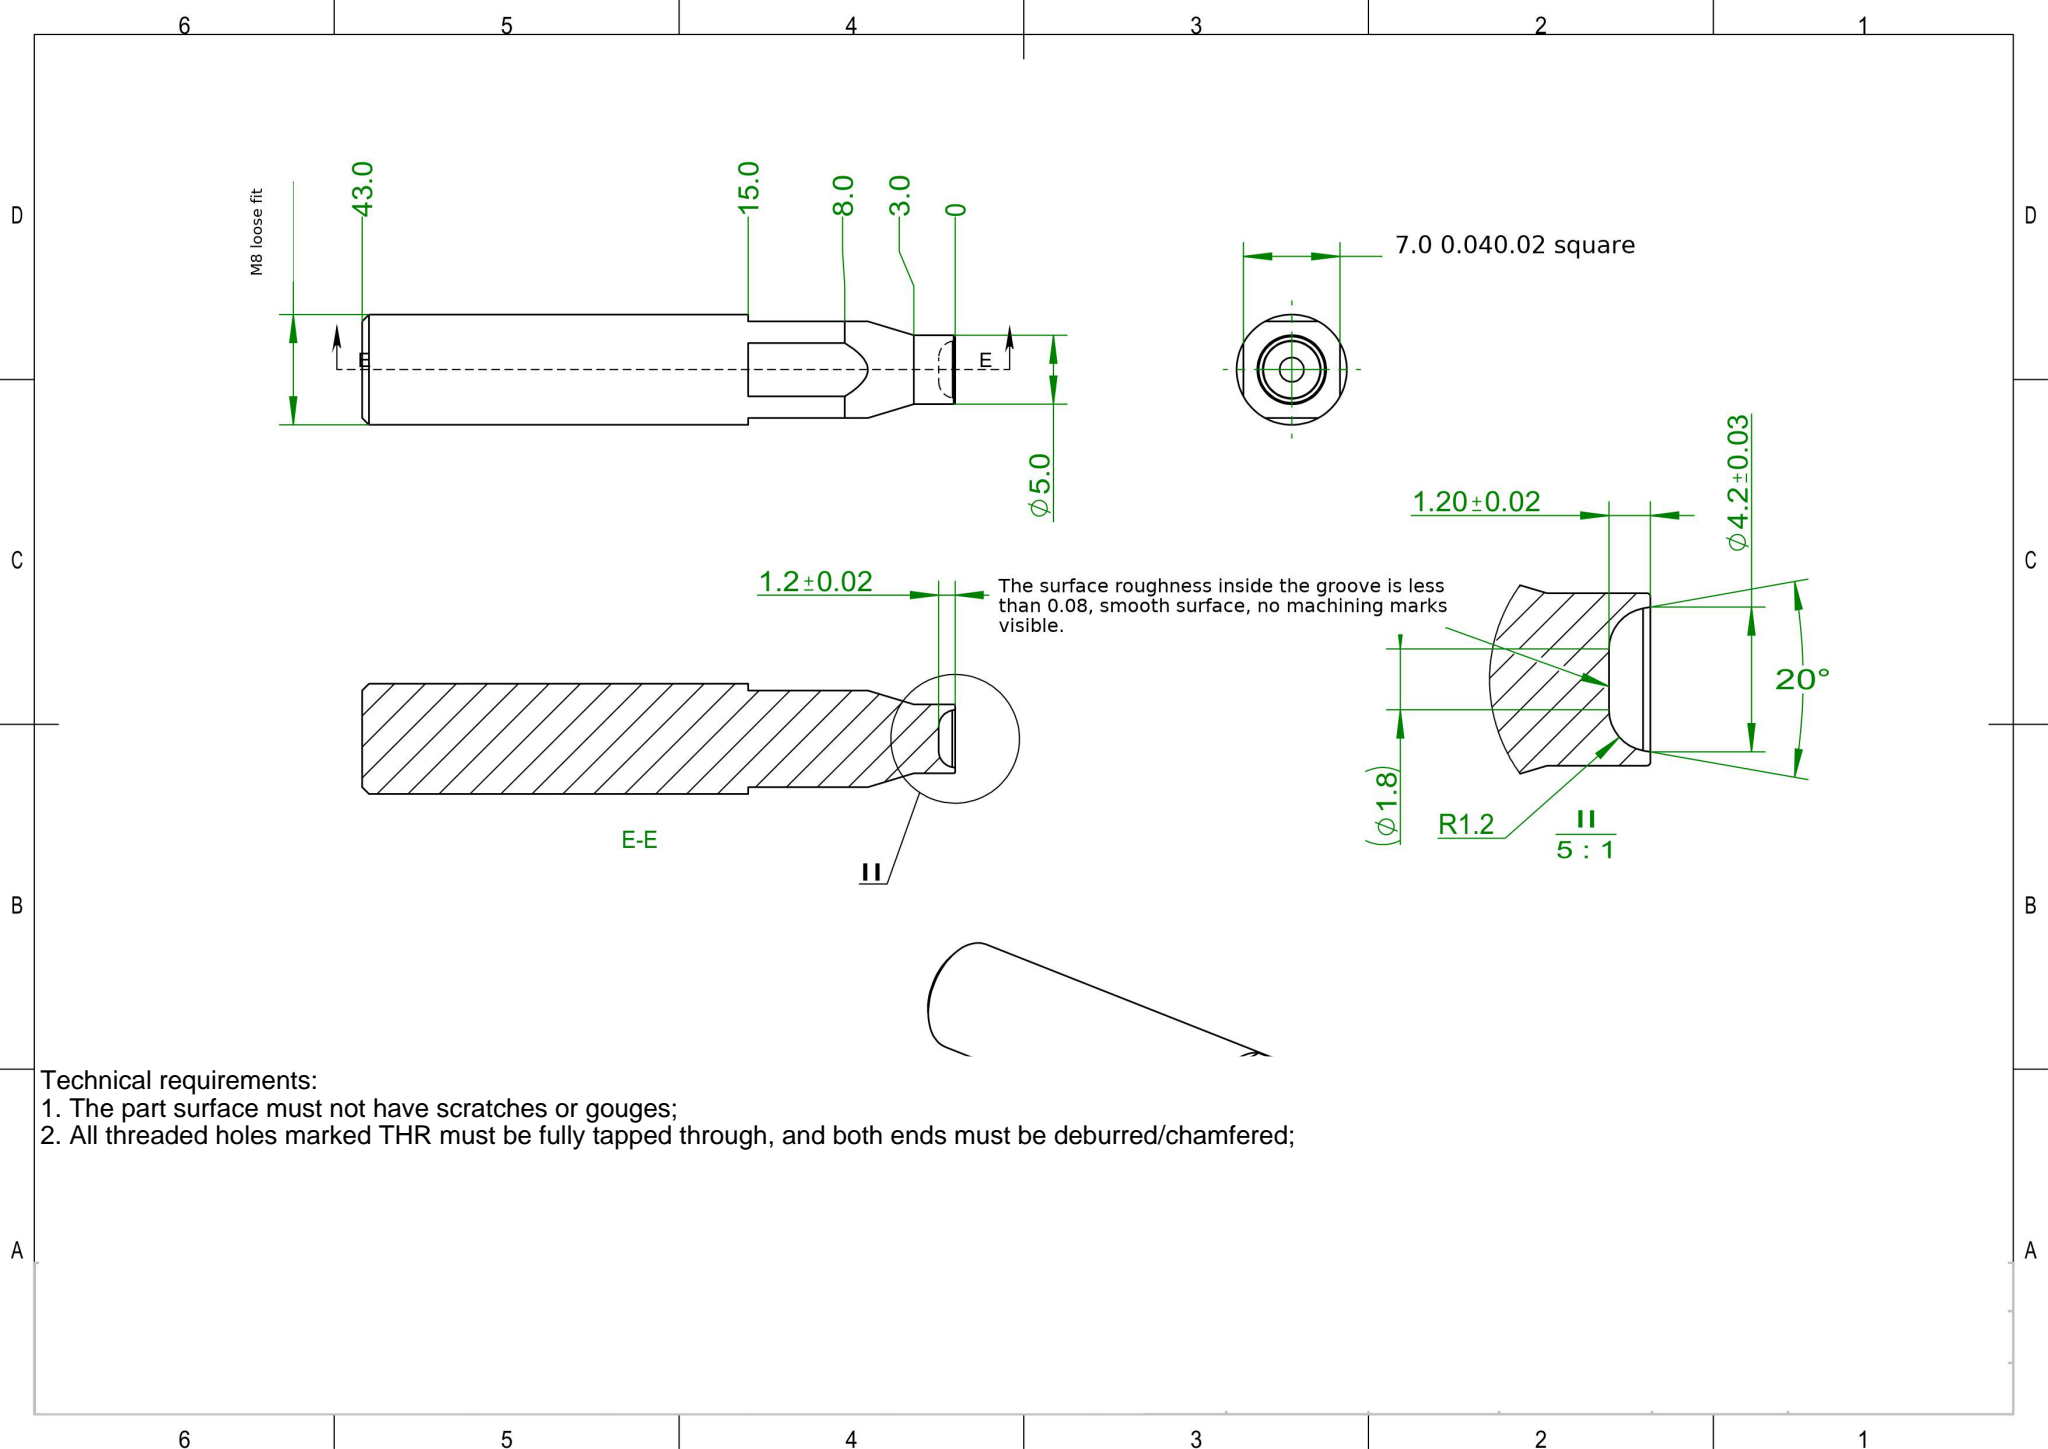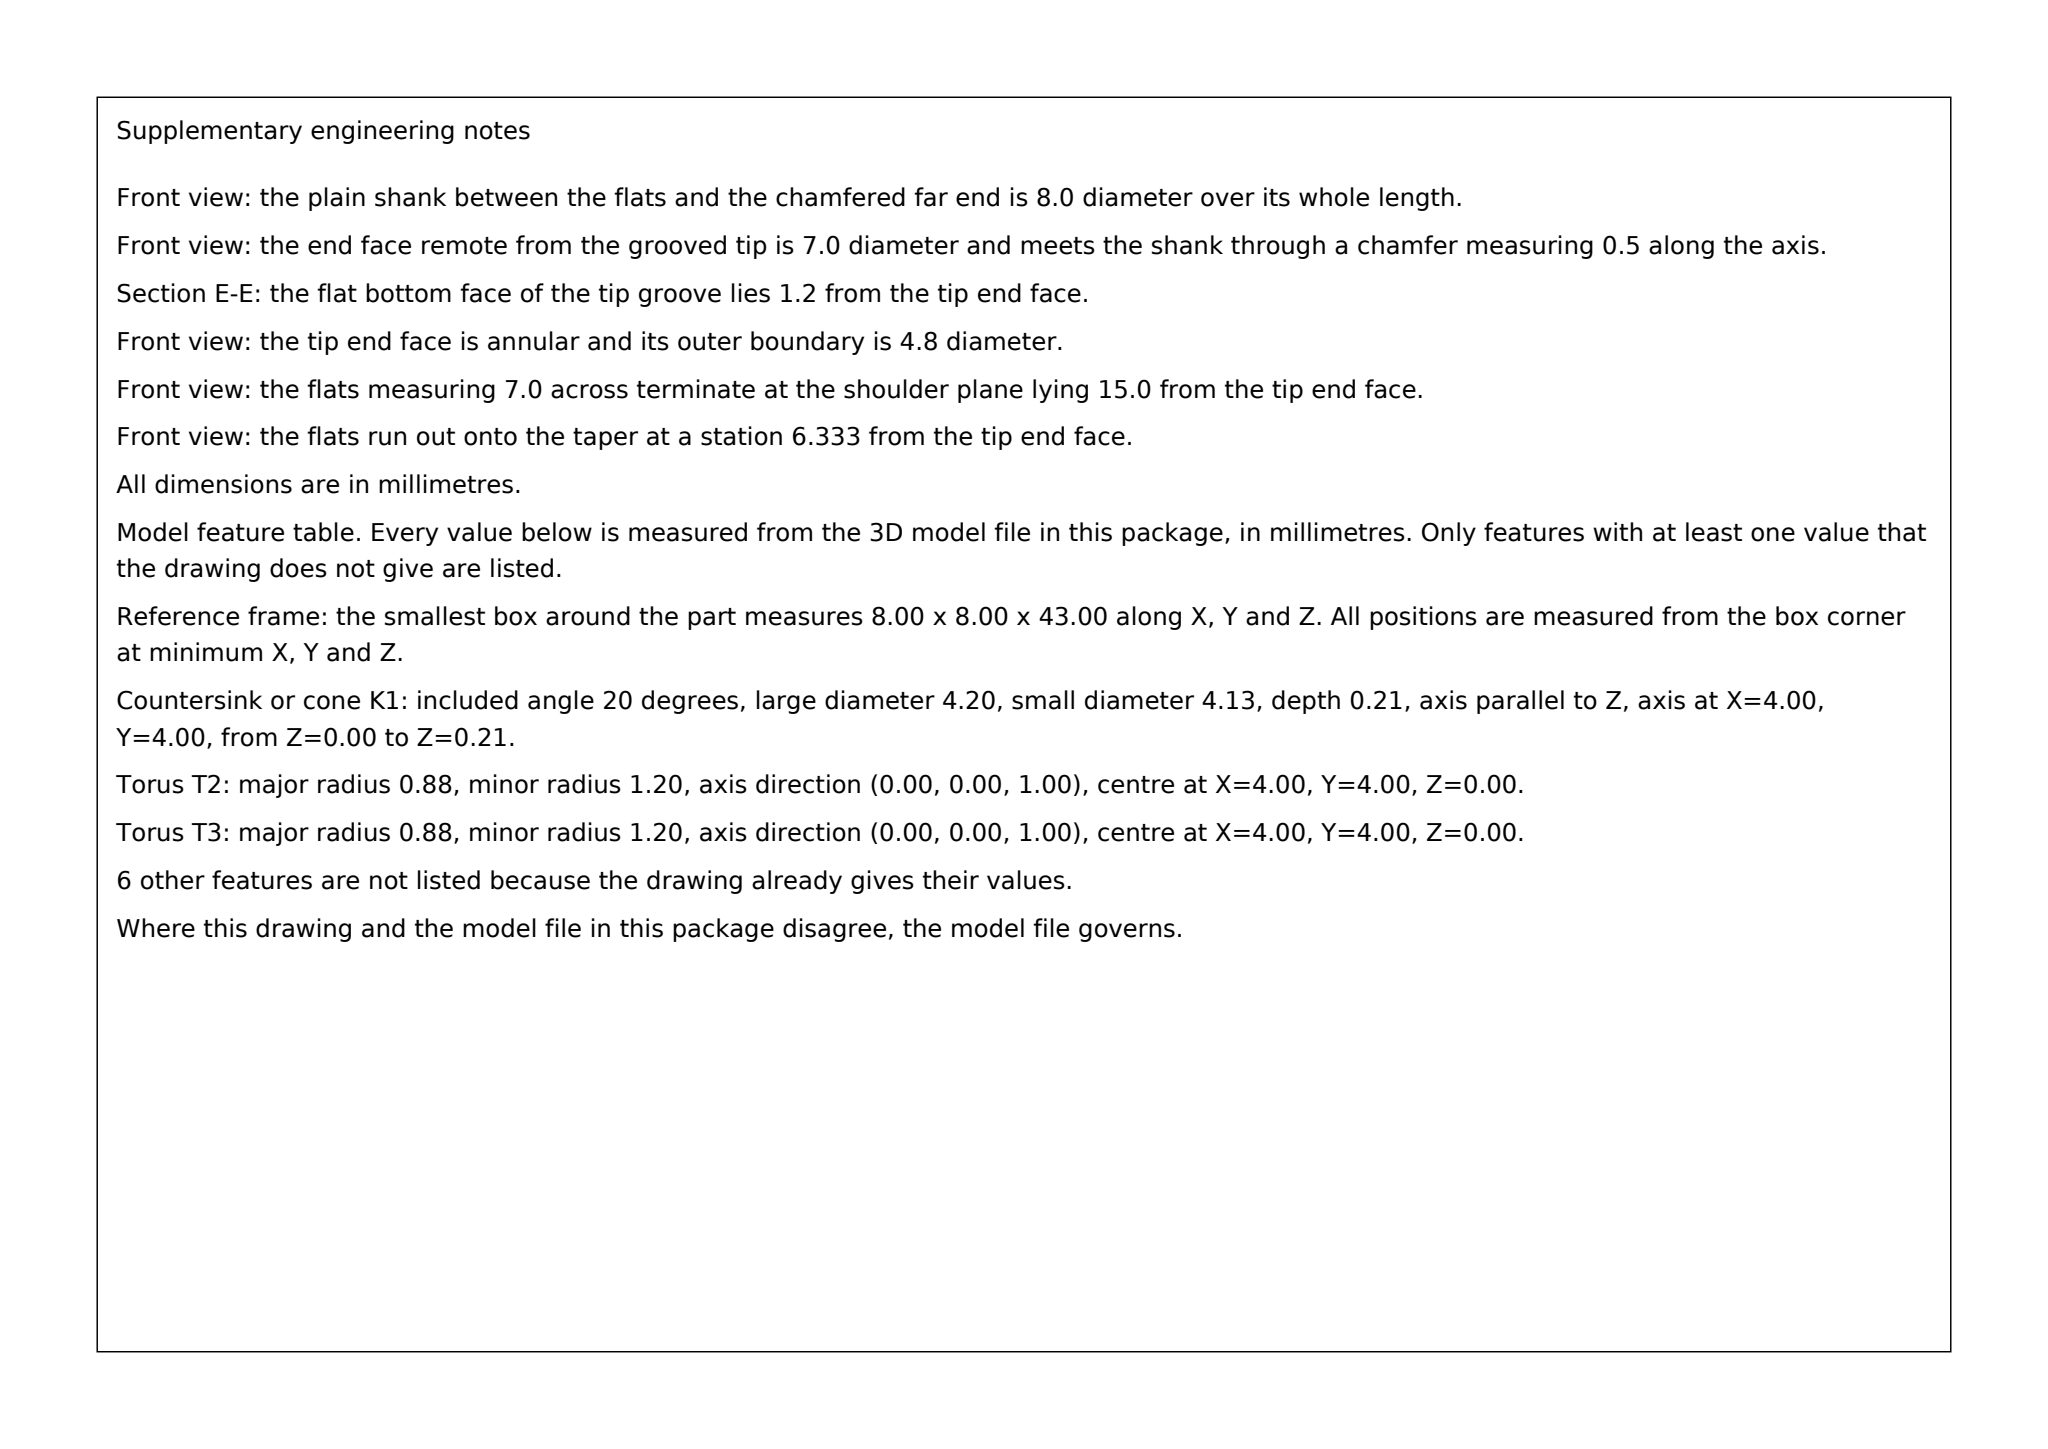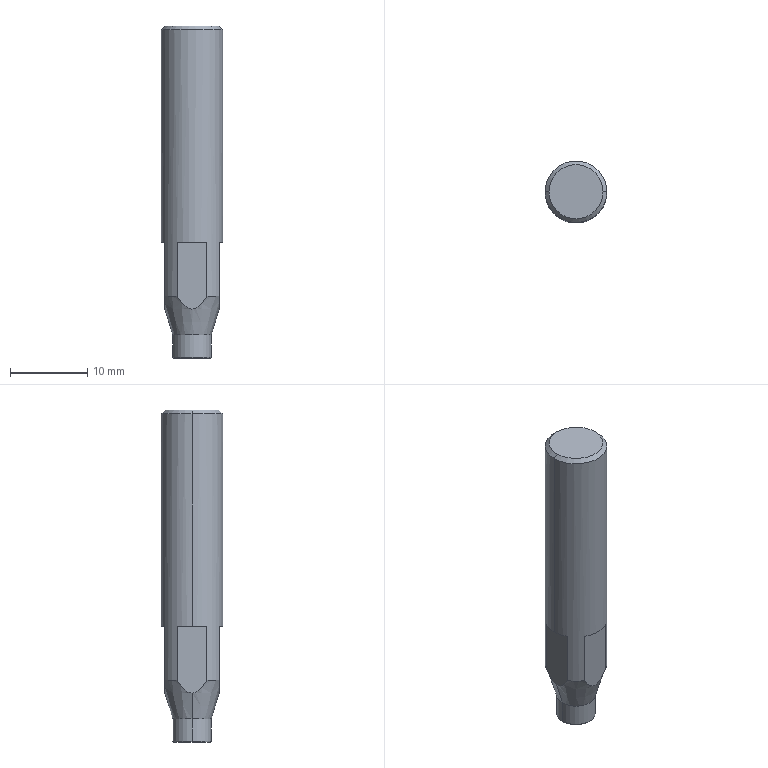Part | SolidWorks | mm | 1 solid | 25 faces | box 8 x 8 x 43 mm | volume 1931 mm3 | plane 11 | cone 6 | torus 4 | cylinder 4 | commonest cylinder face diameters 5 x2 8 x2
Drawing notes:
MAIN BODY OD Ø8.0, ORD 8.0 TO 43.0 (34.5 LG) | from the solid: cylinder [8.0 dia, z axis, 34.5 long] on axis x=4,y=4
TAPER 33.4° INCL, Ø8.0 TO Ø5.0, ORD 8.0 TO 3.0 | from the solid: cone [included 33.4°, ref dia 8.0]; Ø5 and Ø8 cylinders coaxial
R0.1 FILLETS (2) AT Ø5.0 NOSE TRANSITION | from the solid: fillet_radii [0.1, count 2]
DETAIL II: GROOVE FLAT BOT Ø1.76 AT 1.2 DP, BLEND R1.2 | from the solid: Plane z=1.2 (groove bottom) + cone incl 20° ref Ø4.2 at z=0 face + fillet R1.2: Ø4.2-2(1.2)tan10°=Ø3.777 at bottom, less 2x(1.2/tan50°)=2.014 -> Ø1.76 flat (shown Ø1.8 ref)
SQUARE DRIVE FLATS: 7.0 ACROSS FLATS (TWO PAIRS AT 90°), SYMMETRIC ABOUT PART AXIS ON Ø8.0 BODY; FLAT ENDS AT Z=15.0 FROM NOSE END (Z=0) | from the solid: axis_planes x@0.5 & x@7.5, y@0.5 & y@7.5 (8.0 bbox -> 7.0 across flats); axis_planes z@15.0 (4 faces)
SQUARE DRIVE FLAT RUN-OUT: 90° INCLUDED ANGLE CONE, REF Ø7.0, AT FLAT TERMINATION Z=15.0 FROM NOSE END (Z=0), COAXIAL WITH PART AXIS | from the solid: cones[included_angle,ref_dia] = [90.0, 7.0, 2]; axis_planes z offset 15.0 (count 4)
STEP:
#1=CARTESIAN_POINT('',(-2.063,0.,-1.792));
#2=VERTEX_POINT('',#1);
#3=CARTESIAN_POINT('',(2.063,0.,-1.792));
#4=VERTEX_POINT('',#3);
#5=CARTESIAN_POINT('',(0.,0.,-1.792));
#6=DIRECTION('',(0.,0.,1.));
#7=DIRECTION('',(-1.,0.,0.));
#8=AXIS2_PLACEMENT_3D('',#5,#6,#7);
#9=CIRCLE('',#8,2.063);
#10=EDGE_CURVE('',#2,#4,#9,.T.);
#11=ORIENTED_EDGE('',*,*,#10,.F.);
#12=CARTESIAN_POINT('',(-0.8815,0.,-0.8));
#13=VERTEX_POINT('',#12);
#14=CARTESIAN_POINT('',(-0.8815,0.,-2.));
#15=DIRECTION('',(0.,1.,0.));
#16=DIRECTION('',(-1.,0.,0.));
#17=AXIS2_PLACEMENT_3D('',#14,#15,#16);
#18=CIRCLE('',#17,1.2);
#19=EDGE_CURVE('',#2,#13,#18,.T.);
#20=ORIENTED_EDGE('',*,*,#19,.T.);
#21=CARTESIAN_POINT('',(0.8815,0.,-0.8));
#22=VERTEX_POINT('',#21);
#23=CARTESIAN_POINT('',(0.,0.,-0.8));
#24=DIRECTION('',(0.,0.,-1.));
#25=DIRECTION('',(1.,0.,0.));
#26=AXIS2_PLACEMENT_3D('',#23,#24,#25);
#27=CIRCLE('',#26,0.8815);
#28=EDGE_CURVE('',#22,#13,#27,.T.);
#29=ORIENTED_EDGE('',*,*,#28,.F.);
#30=CARTESIAN_POINT('',(0.8815,0.,-2.));
#31=DIRECTION('',(0.,-1.,0.));
#32=DIRECTION('',(0.,0.,-1.));
#33=AXIS2_PLACEMENT_3D('',#30,#31,#32);
#34=CIRCLE('',#33,1.2);
#35=EDGE_CURVE('',#4,#22,#34,.T.);
#36=ORIENTED_EDGE('',*,*,#35,.F.);
#37=EDGE_LOOP('',(#11,#20,#29,#36));
#38=FACE_OUTER_BOUND('',#37,.T.);
#39=CARTESIAN_POINT('',(0.,0.,-2.));
#40=DIRECTION('',(0.,0.,1.));
#41=DIRECTION('',(1.,0.,0.));
#42=AXIS2_PLACEMENT_3D('',#39,#40,#41);
#43=TOROIDAL_SURFACE('',#42,0.8815,1.2);
#44=ADVANCED_FACE('',(#38),#43,.F.);
#45=ORIENTED_EDGE('',*,*,#10,.T.);
#46=CARTESIAN_POINT('',(2.1,0.,-2.));
#47=VERTEX_POINT('',#46);
#48=CARTESIAN_POINT('',(2.1,0.,-2.));
#49=DIRECTION('',(0.1736,0.,-0.9848));
#50=VECTOR('',#49,1000.);
#51=LINE('',#48,#50);
#52=EDGE_CURVE('',#4,#47,#51,.T.);
#53=ORIENTED_EDGE('',*,*,#52,.T.);
#54=CARTESIAN_POINT('',(-2.1,0.,-2.));
#55=VERTEX_POINT('',#54);
#56=CARTESIAN_POINT('',(0.,0.,-2.));
#57=DIRECTION('',(0.,0.,-1.));
#58=DIRECTION('',(-1.,0.,0.));
#59=AXIS2_PLACEMENT_3D('',#56,#57,#58);
#60=CIRCLE('',#59,2.1);
#61=EDGE_CURVE('',#47,#55,#60,.T.);
#62=ORIENTED_EDGE('',*,*,#61,.T.);
#63=CARTESIAN_POINT('',(-2.1,0.,-2.));
#64=DIRECTION('',(-0.1736,0.,-0.9848));
#65=VECTOR('',#64,1000.);
#66=LINE('',#63,#65);
#67=EDGE_CURVE('',#2,#55,#66,.T.);
#68=ORIENTED_EDGE('',*,*,#67,.F.);
#69=EDGE_LOOP('',(#45,#53,#62,#68));
#70=FACE_OUTER_BOUND('',#69,.T.);
#71=CARTESIAN_POINT('',(0.,0.,-2.));
#72=DIRECTION('',(0.,0.,-1.));
#73=DIRECTION('',(-1.,0.,0.));
#74=AXIS2_PLACEMENT_3D('',#71,#72,#73);
#75=CONICAL_SURFACE('',#74,2.1,0.1745);
#76=ADVANCED_FACE('',(#70),#75,.F.);
#77=CARTESIAN_POINT('',(3.5,0.,41.));
#78=VERTEX_POINT('',#77);
#79=CARTESIAN_POINT('',(-3.5,0.,41.));
#80=VERTEX_POINT('',#79);
#81=CARTESIAN_POINT('',(0.,0.,41.));
#82=DIRECTION('',(0.,0.,1.));
#83=DIRECTION('',(1.,0.,0.));
#84=AXIS2_PLACEMENT_3D('',#81,#82,#83);
#85=CIRCLE('',#84,3.5);
#86=EDGE_CURVE('',#78,#80,#85,.T.);
#87=ORIENTED_EDGE('',*,*,#86,.F.);
#88=CARTESIAN_POINT('',(4.,0.,40.5));
#89=VERTEX_POINT('',#88);
#90=CARTESIAN_POINT('',(3.5,0.,41.));
#91=DIRECTION('',(0.7071,0.,-0.7071));
#92=VECTOR('',#91,1000.);
#93=LINE('',#90,#92);
#94=EDGE_CURVE('',#78,#89,#93,.T.);
#95=ORIENTED_EDGE('',*,*,#94,.T.);
#96=CARTESIAN_POINT('',(-4.,0.,40.5));
#97=VERTEX_POINT('',#96);
#98=CARTESIAN_POINT('',(0.,0.,40.5));
#99=DIRECTION('',(0.,0.,-1.));
#100=DIRECTION('',(1.,0.,0.));
#101=AXIS2_PLACEMENT_3D('',#98,#99,#100);
#102=CIRCLE('',#101,4.);
#103=EDGE_CURVE('',#97,#89,#102,.T.);
#104=ORIENTED_EDGE('',*,*,#103,.F.);
#105=CARTESIAN_POINT('',(-3.5,0.,41.));
#106=DIRECTION('',(-0.7071,0.,-0.7071));
#107=VECTOR('',#106,1000.);
#108=LINE('',#105,#107);
#109=EDGE_CURVE('',#80,#97,#108,.T.);
#110=ORIENTED_EDGE('',*,*,#109,.F.);
#111=EDGE_LOOP('',(#87,#95,#104,#110));
#112=FACE_OUTER_BOUND('',#111,.T.);
#113=CARTESIAN_POINT('',(0.,0.,41.));
#114=DIRECTION('',(0.,0.,-1.));
#115=DIRECTION('',(-1.,0.,0.));
#116=AXIS2_PLACEMENT_3D('',#113,#114,#115);
#117=CONICAL_SURFACE('',#116,3.5,0.7854);
#118=ADVANCED_FACE('',(#112),#117,.T.);
#119=CARTESIAN_POINT('',(2.5,0.,1.));
#120=VERTEX_POINT('',#119);
#121=CARTESIAN_POINT('',(-2.5,0.,1.));
#122=VERTEX_POINT('',#121);
#123=CARTESIAN_POINT('',(0.,0.,1.));
#124=DIRECTION('',(0.,0.,1.));
#125=DIRECTION('',(1.,0.,0.));
#126=AXIS2_PLACEMENT_3D('',#123,#124,#125);
#127=CIRCLE('',#126,2.5);
#128=EDGE_CURVE('',#120,#122,#127,.T.);
#129=ORIENTED_EDGE('',*,*,#128,.F.);
#130=CARTESIAN_POINT('',(2.5,0.,-1.9));
#131=VERTEX_POINT('',#130);
#132=CARTESIAN_POINT('',(2.5,0.,11.5));
#133=DIRECTION('',(0.,0.,-1.));
#134=VECTOR('',#133,1000.);
#135=LINE('',#132,#134);
#136=EDGE_CURVE('',#120,#131,#135,.T.);
#137=ORIENTED_EDGE('',*,*,#136,.T.);
#138=CARTESIAN_POINT('',(-2.5,0.,-1.9));
#139=VERTEX_POINT('',#138);
#140=CARTESIAN_POINT('',(0.,0.,-1.9));
#141=DIRECTION('',(0.,0.,1.));
#142=DIRECTION('',(1.,0.,0.));
#143=AXIS2_PLACEMENT_3D('',#140,#141,#142);
#144=CIRCLE('',#143,2.5);
#145=EDGE_CURVE('',#131,#139,#144,.T.);
#146=ORIENTED_EDGE('',*,*,#145,.T.);
#147=CARTESIAN_POINT('',(-2.5,0.,11.5));
#148=DIRECTION('',(0.,0.,-1.));
#149=VECTOR('',#148,1000.);
#150=LINE('',#147,#149);
#151=EDGE_CURVE('',#122,#139,#150,.T.);
#152=ORIENTED_EDGE('',*,*,#151,.F.);
#153=EDGE_LOOP('',(#129,#137,#146,#152));
#154=FACE_OUTER_BOUND('',#153,.T.);
#155=CARTESIAN_POINT('',(0.,0.,11.5));
#156=DIRECTION('',(0.,0.,-1.));
#157=DIRECTION('',(-1.,0.,0.));
#158=AXIS2_PLACEMENT_3D('',#155,#156,#157);
#159=CYLINDRICAL_SURFACE('',#158,2.5);
#160=ADVANCED_FACE('',(#154),#159,.T.);
#161=CARTESIAN_POINT('',(-2.4,0.,-2.));
#162=VERTEX_POINT('',#161);
#163=CARTESIAN_POINT('',(2.4,0.,-2.));
#164=VERTEX_POINT('',#163);
#165=CARTESIAN_POINT('',(0.,0.,-2.));
#166=DIRECTION('',(0.,0.,-1.));
#167=DIRECTION('',(1.,0.,0.));
#168=AXIS2_PLACEMENT_3D('',#165,#166,#167);
#169=CIRCLE('',#168,2.4);
#170=EDGE_CURVE('',#162,#164,#169,.T.);
#171=ORIENTED_EDGE('',*,*,#170,.F.);
#172=CARTESIAN_POINT('',(-2.4,0.,-1.9));
#173=DIRECTION('',(0.,1.,0.));
#174=DIRECTION('',(-1.,0.,0.));
#175=AXIS2_PLACEMENT_3D('',#172,#173,#174);
#176=CIRCLE('',#175,0.1);
#177=EDGE_CURVE('',#162,#139,#176,.T.);
#178=ORIENTED_EDGE('',*,*,#177,.T.);
#179=ORIENTED_EDGE('',*,*,#145,.F.);
#180=CARTESIAN_POINT('',(2.4,0.,-1.9));
#181=DIRECTION('',(0.,-1.,0.));
#182=DIRECTION('',(0.,0.,-1.));
#183=AXIS2_PLACEMENT_3D('',#180,#181,#182);
#184=CIRCLE('',#183,0.1);
#185=EDGE_CURVE('',#164,#131,#184,.T.);
#186=ORIENTED_EDGE('',*,*,#185,.F.);
#187=EDGE_LOOP('',(#171,#178,#179,#186));
#188=FACE_OUTER_BOUND('',#187,.T.);
#189=CARTESIAN_POINT('',(0.,0.,-1.9));
#190=DIRECTION('',(0.,0.,1.));
#191=DIRECTION('',(1.,0.,0.));
#192=AXIS2_PLACEMENT_3D('',#189,#190,#191);
#193=TOROIDAL_SURFACE('',#192,2.4,0.1);
#194=ADVANCED_FACE('',(#188),#193,.T.);
#195=ORIENTED_EDGE('',*,*,#103,.T.);
#196=CARTESIAN_POINT('',(4.,0.,13.));
#197=VERTEX_POINT('',#196);
#198=CARTESIAN_POINT('',(4.,0.,37.814));
#199=DIRECTION('',(0.,0.,-1.));
#200=VECTOR('',#199,1000.);
#201=LINE('',#198,#200);
#202=EDGE_CURVE('',#89,#197,#201,.T.);
#203=ORIENTED_EDGE('',*,*,#202,.T.);
#204=CARTESIAN_POINT('',(3.5,1.936,13.));
#205=VERTEX_POINT('',#204);
#206=CARTESIAN_POINT('',(0.,0.,13.));
#207=DIRECTION('',(0.,0.,1.));
#208=DIRECTION('',(-1.,0.,0.));
#209=AXIS2_PLACEMENT_3D('',#206,#207,#208);
#210=CIRCLE('',#209,4.);
#211=EDGE_CURVE('',#197,#205,#210,.T.);
#212=ORIENTED_EDGE('',*,*,#211,.T.);
#213=CARTESIAN_POINT('',(3.5,1.936,6.));
#214=VERTEX_POINT('',#213);
#215=CARTESIAN_POINT('',(3.5,1.936,15.));
#216=DIRECTION('',(0.,0.,-1.));
#217=VECTOR('',#216,1000.);
#218=LINE('',#215,#217);
#219=EDGE_CURVE('',#205,#214,#218,.T.);
#220=ORIENTED_EDGE('',*,*,#219,.T.);
#221=CARTESIAN_POINT('',(1.936,3.5,6.));
#222=VERTEX_POINT('',#221);
#223=CARTESIAN_POINT('',(0.,0.,6.));
#224=DIRECTION('',(0.,0.,-1.));
#225=DIRECTION('',(1.,0.,0.));
#226=AXIS2_PLACEMENT_3D('',#223,#224,#225);
#227=CIRCLE('',#226,4.);
#228=EDGE_CURVE('',#222,#214,#227,.T.);
#229=ORIENTED_EDGE('',*,*,#228,.F.);
#230=CARTESIAN_POINT('',(1.936,3.5,13.));
#231=VERTEX_POINT('',#230);
#232=CARTESIAN_POINT('',(1.936,3.5,15.));
#233=DIRECTION('',(0.,0.,1.));
#234=VECTOR('',#233,1000.);
#235=LINE('',#232,#234);
#236=EDGE_CURVE('',#222,#231,#235,.T.);
#237=ORIENTED_EDGE('',*,*,#236,.T.);
#238=CARTESIAN_POINT('',(-1.936,3.5,13.));
#239=VERTEX_POINT('',#238);
#240=CARTESIAN_POINT('',(0.,0.,13.));
#241=DIRECTION('',(0.,0.,1.));
#242=DIRECTION('',(-1.,0.,0.));
#243=AXIS2_PLACEMENT_3D('',#240,#241,#242);
#244=CIRCLE('',#243,4.);
#245=EDGE_CURVE('',#231,#239,#244,.T.);
#246=ORIENTED_EDGE('',*,*,#245,.T.);
#247=CARTESIAN_POINT('',(-1.936,3.5,6.));
#248=VERTEX_POINT('',#247);
#249=CARTESIAN_POINT('',(-1.936,3.5,15.));
#250=DIRECTION('',(0.,0.,-1.));
#251=VECTOR('',#250,1000.);
#252=LINE('',#249,#251);
#253=EDGE_CURVE('',#239,#248,#252,.T.);
#254=ORIENTED_EDGE('',*,*,#253,.T.);
#255=CARTESIAN_POINT('',(-3.5,1.936,6.));
#256=VERTEX_POINT('',#255);
#257=CARTESIAN_POINT('',(0.,0.,6.));
#258=DIRECTION('',(0.,0.,-1.));
#259=DIRECTION('',(1.,0.,0.));
#260=AXIS2_PLACEMENT_3D('',#257,#258,#259);
#261=CIRCLE('',#260,4.);
#262=EDGE_CURVE('',#256,#248,#261,.T.);
#263=ORIENTED_EDGE('',*,*,#262,.F.);
#264=CARTESIAN_POINT('',(-3.5,1.936,13.));
#265=VERTEX_POINT('',#264);
#266=CARTESIAN_POINT('',(-3.5,1.936,4.));
#267=DIRECTION('',(0.,0.,1.));
#268=VECTOR('',#267,1000.);
#269=LINE('',#266,#268);
#270=EDGE_CURVE('',#256,#265,#269,.T.);
#271=ORIENTED_EDGE('',*,*,#270,.T.);
#272=CARTESIAN_POINT('',(-4.,0.,13.));
#273=VERTEX_POINT('',#272);
#274=CARTESIAN_POINT('',(0.,0.,13.));
#275=DIRECTION('',(0.,0.,1.));
#276=DIRECTION('',(-1.,0.,0.));
#277=AXIS2_PLACEMENT_3D('',#274,#275,#276);
#278=CIRCLE('',#277,4.);
#279=EDGE_CURVE('',#265,#273,#278,.T.);
#280=ORIENTED_EDGE('',*,*,#279,.T.);
#281=CARTESIAN_POINT('',(-4.,0.,37.814));
#282=DIRECTION('',(0.,0.,-1.));
#283=VECTOR('',#282,1000.);
#284=LINE('',#281,#283);
#285=EDGE_CURVE('',#97,#273,#284,.T.);
#286=ORIENTED_EDGE('',*,*,#285,.F.);
#287=EDGE_LOOP('',(#195,#203,#212,#220,#229,#237,#246,#254,#263,#271,#280,#286));
#288=FACE_OUTER_BOUND('',#287,.T.);
#289=CARTESIAN_POINT('',(0.,0.,37.814));
#290=DIRECTION('',(0.,0.,-1.));
#291=DIRECTION('',(-1.,0.,0.));
#292=AXIS2_PLACEMENT_3D('',#289,#290,#291);
#293=CYLINDRICAL_SURFACE('',#292,4.);
#294=ADVANCED_FACE('',(#288),#293,.T.);
#295=ORIENTED_EDGE('',*,*,#128,.T.);
#296=CARTESIAN_POINT('',(-3.5,0.,4.333));
#297=VERTEX_POINT('',#296);
#298=CARTESIAN_POINT('',(-4.,0.,6.));
#299=DIRECTION('',(-0.2873,0.,0.9578));
#300=VECTOR('',#299,1000.);
#301=LINE('',#298,#300);
#302=EDGE_CURVE('',#122,#297,#301,.T.);
#303=ORIENTED_EDGE('',*,*,#302,.T.);
#304=CARTESIAN_POINT('',(-3.5,0.,4.333));
#305=CARTESIAN_POINT('',(-3.5,0.1104,4.333));
#306=CARTESIAN_POINT('',(-3.5,0.2215,4.351));
#307=CARTESIAN_POINT('',(-3.5,0.4337,4.417));
#308=CARTESIAN_POINT('',(-3.5,0.5339,4.464));
#309=CARTESIAN_POINT('',(-3.5,0.8214,4.634));
#310=CARTESIAN_POINT('',(-3.5,0.9886,4.78));
#311=CARTESIAN_POINT('',(-3.5,1.296,5.098));
#312=CARTESIAN_POINT('',(-3.5,1.436,5.271));
#313=CARTESIAN_POINT('',(-3.5,1.698,5.627));
#314=CARTESIAN_POINT('',(-3.5,1.82,5.812));
#315=CARTESIAN_POINT('',(-3.5,1.936,6.));
#316=B_SPLINE_CURVE_WITH_KNOTS('',3,(#304,#305,#306,#307,#308,#309,#310,#311,#312,#313,#314,#315),.UNSPECIFIED.,.F.,.F.,(4,2,2,2,2,4),(0.002638,0.002968,0.003297,0.003956,0.004614,0.005273),.UNSPECIFIED.);
#317=EDGE_CURVE('',#297,#256,#316,.T.);
#318=ORIENTED_EDGE('',*,*,#317,.T.);
#319=ORIENTED_EDGE('',*,*,#262,.T.);
#320=CARTESIAN_POINT('',(-1.936,3.5,6.));
#321=CARTESIAN_POINT('',(-1.82,3.5,5.812));
#322=CARTESIAN_POINT('',(-1.698,3.5,5.628));
#323=CARTESIAN_POINT('',(-1.438,3.5,5.274));
#324=CARTESIAN_POINT('',(-1.3,3.5,5.103));
#325=CARTESIAN_POINT('',(-0.9938,3.5,4.785));
#326=CARTESIAN_POINT('',(-0.8246,3.5,4.636));
#327=CARTESIAN_POINT('',(-0.5381,3.5,4.466));
#328=CARTESIAN_POINT('',(-0.4361,3.5,4.418));
#329=CARTESIAN_POINT('',(-0.2248,3.5,4.352));
#330=CARTESIAN_POINT('',(-0.1126,3.5,4.334));
#331=CARTESIAN_POINT('',(0.1084,3.5,4.333));
#332=CARTESIAN_POINT('',(0.2196,3.5,4.351));
#333=CARTESIAN_POINT('',(0.4321,3.5,4.417));
#334=CARTESIAN_POINT('',(0.5324,3.5,4.463));
#335=CARTESIAN_POINT('',(0.8203,3.5,4.633));
#336=CARTESIAN_POINT('',(0.9877,3.5,4.779));
#337=CARTESIAN_POINT('',(1.295,3.5,5.097));
#338=CARTESIAN_POINT('',(1.436,3.5,5.27));
#339=CARTESIAN_POINT('',(1.697,3.5,5.627));
#340=CARTESIAN_POINT('',(1.82,3.5,5.811));
#341=CARTESIAN_POINT('',(1.936,3.5,6.));
#342=B_SPLINE_CURVE_WITH_KNOTS('',3,(#320,#321,#322,#323,#324,#325,#326,#327,#328,#329,#330,#331,#332,#333,#334,#335,#336,#337,#338,#339,#340,#341),.UNSPECIFIED.,.F.,.F.,(4,2,2,2,2,2,2,2,2,2,4),(0.,0.0006591,0.001318,0.001977,0.002307,0.002636,0.002966,0.003295,0.003955,0.004614,0.005273),.UNSPECIFIED.);
#343=EDGE_CURVE('',#248,#222,#342,.T.);
#344=ORIENTED_EDGE('',*,*,#343,.T.);
#345=ORIENTED_EDGE('',*,*,#228,.T.);
#346=CARTESIAN_POINT('',(3.5,-0.,4.333));
#347=VERTEX_POINT('',#346);
#348=CARTESIAN_POINT('',(3.5,1.936,6.));
#349=CARTESIAN_POINT('',(3.5,1.82,5.812));
#350=CARTESIAN_POINT('',(3.5,1.698,5.628));
#351=CARTESIAN_POINT('',(3.5,1.438,5.273));
#352=CARTESIAN_POINT('',(3.5,1.3,5.102));
#353=CARTESIAN_POINT('',(3.5,0.993,4.784));
#354=CARTESIAN_POINT('',(3.5,0.8236,4.636));
#355=CARTESIAN_POINT('',(3.5,0.5367,4.466));
#356=CARTESIAN_POINT('',(3.5,0.4345,4.418));
#357=CARTESIAN_POINT('',(3.5,0.2229,4.352));
#358=CARTESIAN_POINT('',(3.5,0.1105,4.333));
#359=CARTESIAN_POINT('',(3.5,-0.,4.333));
#360=B_SPLINE_CURVE_WITH_KNOTS('',3,(#348,#349,#350,#351,#352,#353,#354,#355,#356,#357,#358,#359),.UNSPECIFIED.,.F.,.F.,(4,2,2,2,2,4),(0.,0.0006596,0.001319,0.001979,0.002309,0.002638),.UNSPECIFIED.);
#361=EDGE_CURVE('',#214,#347,#360,.T.);
#362=ORIENTED_EDGE('',*,*,#361,.T.);
#363=CARTESIAN_POINT('',(4.,0.,6.));
#364=DIRECTION('',(0.2873,0.,0.9578));
#365=VECTOR('',#364,1000.);
#366=LINE('',#363,#365);
#367=EDGE_CURVE('',#120,#347,#366,.T.);
#368=ORIENTED_EDGE('',*,*,#367,.F.);
#369=EDGE_LOOP('',(#295,#303,#318,#319,#344,#345,#362,#368));
#370=FACE_OUTER_BOUND('',#369,.T.);
#371=CARTESIAN_POINT('',(0.,0.,6.));
#372=DIRECTION('',(0.,0.,1.));
#373=DIRECTION('',(1.,0.,0.));
#374=AXIS2_PLACEMENT_3D('',#371,#372,#373);
#375=CONICAL_SURFACE('',#374,4.,0.2915);
#376=ADVANCED_FACE('',(#370),#375,.T.);
#377=ORIENTED_EDGE('',*,*,#302,.F.);
#378=CARTESIAN_POINT('',(0.,0.,1.));
#379=DIRECTION('',(0.,0.,1.));
#380=DIRECTION('',(1.,0.,0.));
#381=AXIS2_PLACEMENT_3D('',#378,#379,#380);
#382=CIRCLE('',#381,2.5);
#383=EDGE_CURVE('',#122,#120,#382,.T.);
#384=ORIENTED_EDGE('',*,*,#383,.T.);
#385=ORIENTED_EDGE('',*,*,#367,.T.);
#386=CARTESIAN_POINT('',(3.5,-1.936,6.));
#387=VERTEX_POINT('',#386);
#388=CARTESIAN_POINT('',(3.5,-0.,4.333));
#389=CARTESIAN_POINT('',(3.5,-0.1104,4.333));
#390=CARTESIAN_POINT('',(3.5,-0.2215,4.351));
#391=CARTESIAN_POINT('',(3.5,-0.4337,4.417));
#392=CARTESIAN_POINT('',(3.5,-0.5339,4.464));
#393=CARTESIAN_POINT('',(3.5,-0.8214,4.634));
#394=CARTESIAN_POINT('',(3.5,-0.9886,4.78));
#395=CARTESIAN_POINT('',(3.5,-1.296,5.098));
#396=CARTESIAN_POINT('',(3.5,-1.436,5.271));
#397=CARTESIAN_POINT('',(3.5,-1.698,5.627));
#398=CARTESIAN_POINT('',(3.5,-1.82,5.812));
#399=CARTESIAN_POINT('',(3.5,-1.936,6.));
#400=B_SPLINE_CURVE_WITH_KNOTS('',3,(#388,#389,#390,#391,#392,#393,#394,#395,#396,#397,#398,#399),.UNSPECIFIED.,.F.,.F.,(4,2,2,2,2,4),(0.002638,0.002968,0.003297,0.003956,0.004614,0.005273),.UNSPECIFIED.);
#401=EDGE_CURVE('',#347,#387,#400,.T.);
#402=ORIENTED_EDGE('',*,*,#401,.T.);
#403=CARTESIAN_POINT('',(1.936,-3.5,6.));
#404=VERTEX_POINT('',#403);
#405=CARTESIAN_POINT('',(0.,0.,6.));
#406=DIRECTION('',(0.,0.,-1.));
#407=DIRECTION('',(1.,0.,0.));
#408=AXIS2_PLACEMENT_3D('',#405,#406,#407);
#409=CIRCLE('',#408,4.);
#410=EDGE_CURVE('',#387,#404,#409,.T.);
#411=ORIENTED_EDGE('',*,*,#410,.T.);
#412=CARTESIAN_POINT('',(-1.936,-3.5,6.));
#413=VERTEX_POINT('',#412);
#414=CARTESIAN_POINT('',(1.936,-3.5,6.));
#415=CARTESIAN_POINT('',(1.82,-3.5,5.812));
#416=CARTESIAN_POINT('',(1.698,-3.5,5.628));
#417=CARTESIAN_POINT('',(1.438,-3.5,5.274));
#418=CARTESIAN_POINT('',(1.3,-3.5,5.103));
#419=CARTESIAN_POINT('',(0.9938,-3.5,4.785));
#420=CARTESIAN_POINT('',(0.8246,-3.5,4.636));
#421=CARTESIAN_POINT('',(0.5381,-3.5,4.466));
#422=CARTESIAN_POINT('',(0.4361,-3.5,4.418));
#423=CARTESIAN_POINT('',(0.2248,-3.5,4.352));
#424=CARTESIAN_POINT('',(0.1126,-3.5,4.334));
#425=CARTESIAN_POINT('',(-0.1084,-3.5,4.333));
#426=CARTESIAN_POINT('',(-0.2196,-3.5,4.351));
#427=CARTESIAN_POINT('',(-0.4321,-3.5,4.417));
#428=CARTESIAN_POINT('',(-0.5324,-3.5,4.463));
#429=CARTESIAN_POINT('',(-0.8203,-3.5,4.633));
#430=CARTESIAN_POINT('',(-0.9877,-3.5,4.779));
#431=CARTESIAN_POINT('',(-1.295,-3.5,5.097));
#432=CARTESIAN_POINT('',(-1.436,-3.5,5.27));
#433=CARTESIAN_POINT('',(-1.697,-3.5,5.627));
#434=CARTESIAN_POINT('',(-1.82,-3.5,5.811));
#435=CARTESIAN_POINT('',(-1.936,-3.5,6.));
#436=B_SPLINE_CURVE_WITH_KNOTS('',3,(#414,#415,#416,#417,#418,#419,#420,#421,#422,#423,#424,#425,#426,#427,#428,#429,#430,#431,#432,#433,#434,#435),.UNSPECIFIED.,.F.,.F.,(4,2,2,2,2,2,2,2,2,2,4),(0.,0.0006591,0.001318,0.001977,0.002307,0.002636,0.002966,0.003295,0.003955,0.004614,0.005273),.UNSPECIFIED.);
#437=EDGE_CURVE('',#404,#413,#436,.T.);
#438=ORIENTED_EDGE('',*,*,#437,.T.);
#439=CARTESIAN_POINT('',(-3.5,-1.936,6.));
#440=VERTEX_POINT('',#439);
#441=CARTESIAN_POINT('',(0.,0.,6.));
#442=DIRECTION('',(0.,0.,-1.));
#443=DIRECTION('',(1.,0.,0.));
#444=AXIS2_PLACEMENT_3D('',#441,#442,#443);
#445=CIRCLE('',#444,4.);
#446=EDGE_CURVE('',#413,#440,#445,.T.);
#447=ORIENTED_EDGE('',*,*,#446,.T.);
#448=CARTESIAN_POINT('',(-3.5,-1.936,6.));
#449=CARTESIAN_POINT('',(-3.5,-1.82,5.812));
#450=CARTESIAN_POINT('',(-3.5,-1.698,5.628));
#451=CARTESIAN_POINT('',(-3.5,-1.438,5.273));
#452=CARTESIAN_POINT('',(-3.5,-1.3,5.102));
#453=CARTESIAN_POINT('',(-3.5,-0.993,4.784));
#454=CARTESIAN_POINT('',(-3.5,-0.8236,4.636));
#455=CARTESIAN_POINT('',(-3.5,-0.5367,4.466));
#456=CARTESIAN_POINT('',(-3.5,-0.4345,4.418));
#457=CARTESIAN_POINT('',(-3.5,-0.2229,4.352));
#458=CARTESIAN_POINT('',(-3.5,-0.1105,4.333));
#459=CARTESIAN_POINT('',(-3.5,0.,4.333));
#460=B_SPLINE_CURVE_WITH_KNOTS('',3,(#448,#449,#450,#451,#452,#453,#454,#455,#456,#457,#458,#459),.UNSPECIFIED.,.F.,.F.,(4,2,2,2,2,4),(0.,0.0006596,0.001319,0.001979,0.002309,0.002638),.UNSPECIFIED.);
#461=EDGE_CURVE('',#440,#297,#460,.T.);
#462=ORIENTED_EDGE('',*,*,#461,.T.);
#463=EDGE_LOOP('',(#377,#384,#385,#402,#411,#438,#447,#462));
#464=FACE_OUTER_BOUND('',#463,.T.);
#465=CARTESIAN_POINT('',(0.,0.,6.));
#466=DIRECTION('',(0.,0.,1.));
#467=DIRECTION('',(1.,0.,0.));
#468=AXIS2_PLACEMENT_3D('',#465,#466,#467);
#469=CONICAL_SURFACE('',#468,4.,0.2915);
#470=ADVANCED_FACE('',(#464),#469,.T.);
#471=ORIENTED_EDGE('',*,*,#202,.F.);
#472=CARTESIAN_POINT('',(0.,0.,40.5));
#473=DIRECTION('',(0.,0.,-1.));
#474=DIRECTION('',(1.,0.,0.));
#475=AXIS2_PLACEMENT_3D('',#472,#473,#474);
#476=CIRCLE('',#475,4.);
#477=EDGE_CURVE('',#89,#97,#476,.T.);
#478=ORIENTED_EDGE('',*,*,#477,.T.);
#479=ORIENTED_EDGE('',*,*,#285,.T.);
#480=CARTESIAN_POINT('',(-3.5,-1.936,13.));
#481=VERTEX_POINT('',#480);
#482=CARTESIAN_POINT('',(0.,0.,13.));
#483=DIRECTION('',(0.,0.,1.));
#484=DIRECTION('',(-1.,0.,0.));
#485=AXIS2_PLACEMENT_3D('',#482,#483,#484);
#486=CIRCLE('',#485,4.);
#487=EDGE_CURVE('',#273,#481,#486,.T.);
#488=ORIENTED_EDGE('',*,*,#487,.T.);
#489=CARTESIAN_POINT('',(-3.5,-1.936,15.));
#490=DIRECTION('',(0.,0.,-1.));
#491=VECTOR('',#490,1000.);
#492=LINE('',#489,#491);
#493=EDGE_CURVE('',#481,#440,#492,.T.);
#494=ORIENTED_EDGE('',*,*,#493,.T.);
#495=ORIENTED_EDGE('',*,*,#446,.F.);
#496=CARTESIAN_POINT('',(-1.936,-3.5,13.));
#497=VERTEX_POINT('',#496);
#498=CARTESIAN_POINT('',(-1.936,-3.5,15.));
#499=DIRECTION('',(0.,0.,1.));
#500=VECTOR('',#499,1000.);
#501=LINE('',#498,#500);
#502=EDGE_CURVE('',#413,#497,#501,.T.);
#503=ORIENTED_EDGE('',*,*,#502,.T.);
#504=CARTESIAN_POINT('',(1.936,-3.5,13.));
#505=VERTEX_POINT('',#504);
#506=CARTESIAN_POINT('',(0.,0.,13.));
#507=DIRECTION('',(0.,0.,1.));
#508=DIRECTION('',(-1.,0.,0.));
#509=AXIS2_PLACEMENT_3D('',#506,#507,#508);
#510=CIRCLE('',#509,4.);
#511=EDGE_CURVE('',#497,#505,#510,.T.);
#512=ORIENTED_EDGE('',*,*,#511,.T.);
#513=CARTESIAN_POINT('',(1.936,-3.5,15.));
#514=DIRECTION('',(0.,0.,-1.));
#515=VECTOR('',#514,1000.);
#516=LINE('',#513,#515);
#517=EDGE_CURVE('',#505,#404,#516,.T.);
#518=ORIENTED_EDGE('',*,*,#517,.T.);
#519=ORIENTED_EDGE('',*,*,#410,.F.);
#520=CARTESIAN_POINT('',(3.5,-1.936,13.));
#521=VERTEX_POINT('',#520);
#522=CARTESIAN_POINT('',(3.5,-1.936,15.));
#523=DIRECTION('',(0.,0.,1.));
#524=VECTOR('',#523,1000.);
#525=LINE('',#522,#524);
#526=EDGE_CURVE('',#387,#521,#525,.T.);
#527=ORIENTED_EDGE('',*,*,#526,.T.);
#528=CARTESIAN_POINT('',(0.,0.,13.));
#529=DIRECTION('',(0.,0.,1.));
#530=DIRECTION('',(-1.,0.,0.));
#531=AXIS2_PLACEMENT_3D('',#528,#529,#530);
#532=CIRCLE('',#531,4.);
#533=EDGE_CURVE('',#521,#197,#532,.T.);
#534=ORIENTED_EDGE('',*,*,#533,.T.);
#535=EDGE_LOOP('',(#471,#478,#479,#488,#494,#495,#503,#512,#518,#519,#527,#534));
#536=FACE_OUTER_BOUND('',#535,.T.);
#537=CARTESIAN_POINT('',(0.,0.,37.814));
#538=DIRECTION('',(0.,0.,-1.));
#539=DIRECTION('',(-1.,0.,0.));
#540=AXIS2_PLACEMENT_3D('',#537,#538,#539);
#541=CYLINDRICAL_SURFACE('',#540,4.);
#542=ADVANCED_FACE('',(#536),#541,.T.);
#543=CARTESIAN_POINT('',(0.,0.,-2.));
#544=DIRECTION('',(0.,0.,-1.));
#545=DIRECTION('',(-1.,0.,0.));
#546=AXIS2_PLACEMENT_3D('',#543,#544,#545);
#547=CIRCLE('',#546,2.1);
#548=EDGE_CURVE('',#55,#47,#547,.T.);
#549=ORIENTED_EDGE('',*,*,#548,.F.);
#550=ORIENTED_EDGE('',*,*,#61,.F.);
#551=EDGE_LOOP('',(#549,#550));
#552=FACE_BOUND('',#551,.T.);
#553=CARTESIAN_POINT('',(0.,0.,-2.));
#554=DIRECTION('',(0.,0.,-1.));
#555=DIRECTION('',(1.,0.,0.));
#556=AXIS2_PLACEMENT_3D('',#553,#554,#555);
#557=CIRCLE('',#556,2.4);
#558=EDGE_CURVE('',#164,#162,#557,.T.);
#559=ORIENTED_EDGE('',*,*,#558,.T.);
#560=ORIENTED_EDGE('',*,*,#170,.T.);
#561=EDGE_LOOP('',(#559,#560));
#562=FACE_OUTER_BOUND('',#561,.T.);
#563=CARTESIAN_POINT('',(0.,-0.,-2.));
#564=DIRECTION('',(0.,0.,1.));
#565=DIRECTION('',(1.,0.,0.));
#566=AXIS2_PLACEMENT_3D('',#563,#564,#565);
#567=PLANE('',#566);
#568=ADVANCED_FACE('',(#552,#562),#567,.F.);
#569=ORIENTED_EDGE('',*,*,#177,.F.);
#570=ORIENTED_EDGE('',*,*,#558,.F.);
#571=ORIENTED_EDGE('',*,*,#185,.T.);
#572=CARTESIAN_POINT('',(0.,0.,-1.9));
#573=DIRECTION('',(0.,0.,1.));
#574=DIRECTION('',(1.,0.,0.));
#575=AXIS2_PLACEMENT_3D('',#572,#573,#574);
#576=CIRCLE('',#575,2.5);
#577=EDGE_CURVE('',#139,#131,#576,.T.);
#578=ORIENTED_EDGE('',*,*,#577,.F.);
#579=EDGE_LOOP('',(#569,#570,#571,#578));
#580=FACE_OUTER_BOUND('',#579,.T.);
#581=CARTESIAN_POINT('',(0.,0.,-1.9));
#582=DIRECTION('',(0.,0.,1.));
#583=DIRECTION('',(1.,0.,0.));
#584=AXIS2_PLACEMENT_3D('',#581,#582,#583);
#585=TOROIDAL_SURFACE('',#584,2.4,0.1);
#586=ADVANCED_FACE('',(#580),#585,.T.);
#587=ORIENTED_EDGE('',*,*,#136,.F.);
#588=ORIENTED_EDGE('',*,*,#383,.F.);
#589=ORIENTED_EDGE('',*,*,#151,.T.);
#590=ORIENTED_EDGE('',*,*,#577,.T.);
#591=EDGE_LOOP('',(#587,#588,#589,#590));
#592=FACE_OUTER_BOUND('',#591,.T.);
#593=CARTESIAN_POINT('',(0.,0.,11.5));
#594=DIRECTION('',(0.,0.,-1.));
#595=DIRECTION('',(-1.,0.,0.));
#596=AXIS2_PLACEMENT_3D('',#593,#594,#595);
#597=CYLINDRICAL_SURFACE('',#596,2.5);
#598=ADVANCED_FACE('',(#592),#597,.T.);
#599=ORIENTED_EDGE('',*,*,#343,.F.);
#600=ORIENTED_EDGE('',*,*,#253,.F.);
#601=CARTESIAN_POINT('',(3.5,3.5,13.));
#602=DIRECTION('',(1.,0.,0.));
#603=VECTOR('',#602,1000.);
#604=LINE('',#601,#603);
#605=EDGE_CURVE('',#239,#231,#604,.T.);
#606=ORIENTED_EDGE('',*,*,#605,.T.);
#607=ORIENTED_EDGE('',*,*,#236,.F.);
#608=EDGE_LOOP('',(#599,#600,#606,#607));
#609=FACE_OUTER_BOUND('',#608,.T.);
#610=CARTESIAN_POINT('',(3.5,3.5,8.));
#611=DIRECTION('',(0.,1.,0.));
#612=DIRECTION('',(0.,0.,1.));
#613=AXIS2_PLACEMENT_3D('',#610,#611,#612);
#614=PLANE('',#613);
#615=ADVANCED_FACE('',(#609),#614,.T.);
#616=ORIENTED_EDGE('',*,*,#605,.F.);
#617=ORIENTED_EDGE('',*,*,#245,.F.);
#618=EDGE_LOOP('',(#616,#617));
#619=FACE_OUTER_BOUND('',#618,.T.);
#620=CARTESIAN_POINT('',(0.,0.,13.));
#621=DIRECTION('',(0.,0.,-1.));
#622=DIRECTION('',(-1.,0.,0.));
#623=AXIS2_PLACEMENT_3D('',#620,#621,#622);
#624=PLANE('',#623);
#625=ADVANCED_FACE('',(#619),#624,.T.);
#626=ORIENTED_EDGE('',*,*,#361,.F.);
#627=ORIENTED_EDGE('',*,*,#219,.F.);
#628=CARTESIAN_POINT('',(3.5,3.5,13.));
#629=DIRECTION('',(-0.,-1.,0.));
#630=VECTOR('',#629,1000.);
#631=LINE('',#628,#630);
#632=EDGE_CURVE('',#205,#521,#631,.T.);
#633=ORIENTED_EDGE('',*,*,#632,.T.);
#634=ORIENTED_EDGE('',*,*,#526,.F.);
#635=ORIENTED_EDGE('',*,*,#401,.F.);
#636=EDGE_LOOP('',(#626,#627,#633,#634,#635));
#637=FACE_OUTER_BOUND('',#636,.T.);
#638=CARTESIAN_POINT('',(3.5,3.5,8.));
#639=DIRECTION('',(1.,-0.,0.));
#640=DIRECTION('',(0.,1.,0.));
#641=AXIS2_PLACEMENT_3D('',#638,#639,#640);
#642=PLANE('',#641);
#643=ADVANCED_FACE('',(#637),#642,.T.);
#644=ORIENTED_EDGE('',*,*,#632,.F.);
#645=ORIENTED_EDGE('',*,*,#211,.F.);
#646=ORIENTED_EDGE('',*,*,#533,.F.);
#647=EDGE_LOOP('',(#644,#645,#646));
#648=FACE_OUTER_BOUND('',#647,.T.);
#649=CARTESIAN_POINT('',(0.,0.,13.));
#650=DIRECTION('',(0.,0.,-1.));
#651=DIRECTION('',(-1.,0.,0.));
#652=AXIS2_PLACEMENT_3D('',#649,#650,#651);
#653=PLANE('',#652);
#654=ADVANCED_FACE('',(#648),#653,.T.);
#655=ORIENTED_EDGE('',*,*,#437,.F.);
#656=ORIENTED_EDGE('',*,*,#517,.F.);
#657=CARTESIAN_POINT('',(3.5,-3.5,13.));
#658=DIRECTION('',(-1.,0.,0.));
#659=VECTOR('',#658,1000.);
#660=LINE('',#657,#659);
#661=EDGE_CURVE('',#505,#497,#660,.T.);
#662=ORIENTED_EDGE('',*,*,#661,.T.);
#663=ORIENTED_EDGE('',*,*,#502,.F.);
#664=EDGE_LOOP('',(#655,#656,#662,#663));
#665=FACE_OUTER_BOUND('',#664,.T.);
#666=CARTESIAN_POINT('',(3.5,-3.5,8.));
#667=DIRECTION('',(0.,-1.,0.));
#668=DIRECTION('',(0.,0.,-1.));
#669=AXIS2_PLACEMENT_3D('',#666,#667,#668);
#670=PLANE('',#669);
#671=ADVANCED_FACE('',(#665),#670,.T.);
#672=ORIENTED_EDGE('',*,*,#661,.F.);
#673=ORIENTED_EDGE('',*,*,#511,.F.);
#674=EDGE_LOOP('',(#672,#673));
#675=FACE_OUTER_BOUND('',#674,.T.);
#676=CARTESIAN_POINT('',(0.,0.,13.));
#677=DIRECTION('',(0.,0.,-1.));
#678=DIRECTION('',(-1.,0.,0.));
#679=AXIS2_PLACEMENT_3D('',#676,#677,#678);
#680=PLANE('',#679);
#681=ADVANCED_FACE('',(#675),#680,.T.);
#682=CARTESIAN_POINT('',(-3.5,3.5,13.));
#683=DIRECTION('',(-0.,1.,0.));
#684=VECTOR('',#683,1000.);
#685=LINE('',#682,#684);
#686=EDGE_CURVE('',#481,#265,#685,.T.);
#687=ORIENTED_EDGE('',*,*,#686,.F.);
#688=ORIENTED_EDGE('',*,*,#487,.F.);
#689=ORIENTED_EDGE('',*,*,#279,.F.);
#690=EDGE_LOOP('',(#687,#688,#689));
#691=FACE_OUTER_BOUND('',#690,.T.);
#692=CARTESIAN_POINT('',(0.,0.,13.));
#693=DIRECTION('',(0.,0.,-1.));
#694=DIRECTION('',(-1.,0.,0.));
#695=AXIS2_PLACEMENT_3D('',#692,#693,#694);
#696=PLANE('',#695);
#697=ADVANCED_FACE('',(#691),#696,.T.);
#698=ORIENTED_EDGE('',*,*,#461,.F.);
#699=ORIENTED_EDGE('',*,*,#493,.F.);
#700=ORIENTED_EDGE('',*,*,#686,.T.);
#701=ORIENTED_EDGE('',*,*,#270,.F.);
#702=ORIENTED_EDGE('',*,*,#317,.F.);
#703=EDGE_LOOP('',(#698,#699,#700,#701,#702));
#704=FACE_OUTER_BOUND('',#703,.T.);
#705=CARTESIAN_POINT('',(-3.5,3.5,8.));
#706=DIRECTION('',(-1.,-0.,0.));
#707=DIRECTION('',(0.,-1.,0.));
#708=AXIS2_PLACEMENT_3D('',#705,#706,#707);
#709=PLANE('',#708);
#710=ADVANCED_FACE('',(#704),#709,.T.);
#711=CARTESIAN_POINT('',(0.,0.,41.));
#712=DIRECTION('',(0.,0.,1.));
#713=DIRECTION('',(1.,0.,0.));
#714=AXIS2_PLACEMENT_3D('',#711,#712,#713);
#715=CIRCLE('',#714,3.5);
#716=EDGE_CURVE('',#80,#78,#715,.T.);
#717=ORIENTED_EDGE('',*,*,#716,.T.);
#718=ORIENTED_EDGE('',*,*,#86,.T.);
#719=EDGE_LOOP('',(#717,#718));
#720=FACE_OUTER_BOUND('',#719,.T.);
#721=CARTESIAN_POINT('',(0.,0.,41.));
#722=DIRECTION('',(0.,0.,1.));
#723=DIRECTION('',(1.,0.,0.));
#724=AXIS2_PLACEMENT_3D('',#721,#722,#723);
#725=PLANE('',#724);
#726=ADVANCED_FACE('',(#720),#725,.T.);
#727=ORIENTED_EDGE('',*,*,#94,.F.);
#728=ORIENTED_EDGE('',*,*,#716,.F.);
#729=ORIENTED_EDGE('',*,*,#109,.T.);
#730=ORIENTED_EDGE('',*,*,#477,.F.);
#731=EDGE_LOOP('',(#727,#728,#729,#730));
#732=FACE_OUTER_BOUND('',#731,.T.);
#733=CARTESIAN_POINT('',(0.,0.,41.));
#734=DIRECTION('',(0.,0.,-1.));
#735=DIRECTION('',(-1.,0.,0.));
#736=AXIS2_PLACEMENT_3D('',#733,#734,#735);
#737=CONICAL_SURFACE('',#736,3.5,0.7854);
#738=ADVANCED_FACE('',(#732),#737,.T.);
#739=ORIENTED_EDGE('',*,*,#52,.F.);
#740=CARTESIAN_POINT('',(0.,0.,-1.792));
#741=DIRECTION('',(0.,0.,1.));
#742=DIRECTION('',(-1.,0.,0.));
#743=AXIS2_PLACEMENT_3D('',#740,#741,#742);
#744=CIRCLE('',#743,2.063);
#745=EDGE_CURVE('',#4,#2,#744,.T.);
#746=ORIENTED_EDGE('',*,*,#745,.T.);
#747=ORIENTED_EDGE('',*,*,#67,.T.);
#748=ORIENTED_EDGE('',*,*,#548,.T.);
#749=EDGE_LOOP('',(#739,#746,#747,#748));
#750=FACE_OUTER_BOUND('',#749,.T.);
#751=CARTESIAN_POINT('',(0.,0.,-2.));
#752=DIRECTION('',(0.,0.,-1.));
#753=DIRECTION('',(-1.,0.,0.));
#754=AXIS2_PLACEMENT_3D('',#751,#752,#753);
#755=CONICAL_SURFACE('',#754,2.1,0.1745);
#756=ADVANCED_FACE('',(#750),#755,.F.);
#757=ORIENTED_EDGE('',*,*,#28,.T.);
#758=CARTESIAN_POINT('',(0.,0.,-0.8));
#759=DIRECTION('',(0.,0.,-1.));
#760=DIRECTION('',(1.,0.,0.));
#761=AXIS2_PLACEMENT_3D('',#758,#759,#760);
#762=CIRCLE('',#761,0.8815);
#763=EDGE_CURVE('',#13,#22,#762,.T.);
#764=ORIENTED_EDGE('',*,*,#763,.T.);
#765=EDGE_LOOP('',(#757,#764));
#766=FACE_OUTER_BOUND('',#765,.T.);
#767=CARTESIAN_POINT('',(0.,0.,-0.8));
#768=DIRECTION('',(0.,0.,1.));
#769=DIRECTION('',(-0.383,0.9237,0.));
#770=AXIS2_PLACEMENT_3D('',#767,#768,#769);
#771=PLANE('',#770);
#772=ADVANCED_FACE('',(#766),#771,.F.);
#773=ORIENTED_EDGE('',*,*,#19,.F.);
#774=ORIENTED_EDGE('',*,*,#745,.F.);
#775=ORIENTED_EDGE('',*,*,#35,.T.);
#776=ORIENTED_EDGE('',*,*,#763,.F.);
#777=EDGE_LOOP('',(#773,#774,#775,#776));
#778=FACE_OUTER_BOUND('',#777,.T.);
#779=CARTESIAN_POINT('',(0.,0.,-2.));
#780=DIRECTION('',(0.,0.,1.));
#781=DIRECTION('',(1.,0.,0.));
#782=AXIS2_PLACEMENT_3D('',#779,#780,#781);
#783=TOROIDAL_SURFACE('',#782,0.8815,1.2);
#784=ADVANCED_FACE('',(#778),#783,.F.);
#785=CLOSED_SHELL('',(#44,#76,#118,#160,#194,#294,#376,#470,#542,#568,#586,#598,#615,#625,#643,#654,#671,#681,#697,#710,#726,#738,#756,#772,#784));
#786=MANIFOLD_SOLID_BREP('',#785);
#787=CARTESIAN_POINT('',(0.,0.,0.));
#788=DIRECTION('',(0.,0.,1.));
#789=DIRECTION('',(1.,0.,0.));
#790=AXIS2_PLACEMENT_3D('',#787,#788,#789);
#791=(LENGTH_UNIT()NAMED_UNIT(*)SI_UNIT(.MILLI.,.METRE.));
#792=UNCERTAINTY_MEASURE_WITH_UNIT(LENGTH_MEASURE(0.00001),#791,'','');
#793=(NAMED_UNIT(*)PLANE_ANGLE_UNIT()SI_UNIT($,.RADIAN.));
#794=(NAMED_UNIT(*)SI_UNIT($,.STERADIAN.)SOLID_ANGLE_UNIT());
#795=(GEOMETRIC_REPRESENTATION_CONTEXT(3)GLOBAL_UNCERTAINTY_ASSIGNED_CONTEXT((#792))GLOBAL_UNIT_ASSIGNED_CONTEXT((#791,#793,#794))REPRESENTATION_CONTEXT('',''));
#796=ADVANCED_BREP_SHAPE_REPRESENTATION('',(#786,#790),#795);